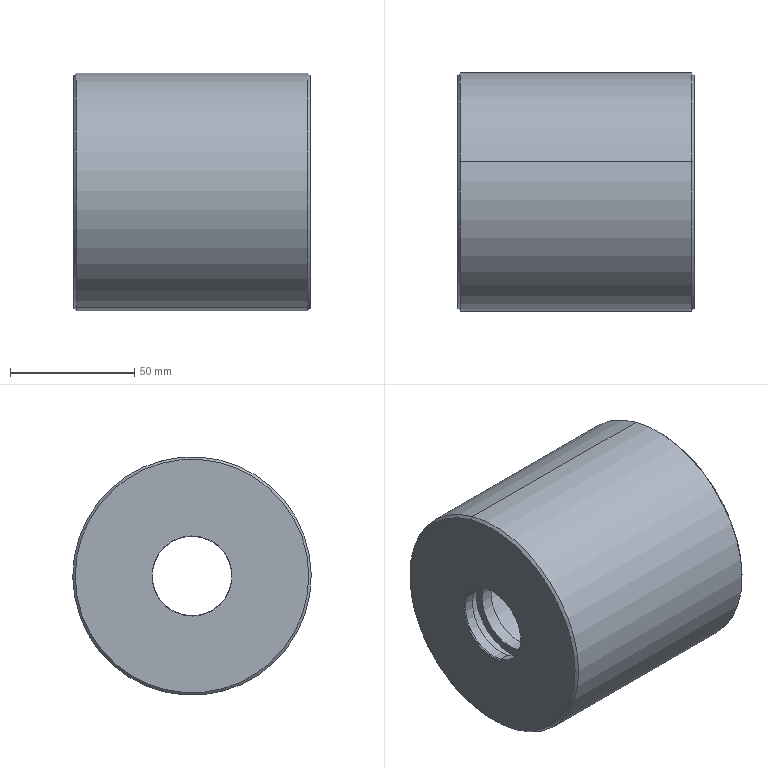Component | SolidWorks | 216InnerTubeAssembly-1_BearingSleeve1-1 | 1 solid | 37 faces | box 95 x 96 x 96 mm | volume 345909 mm3 | cylinder 18 | plane 9 | cone 8 | torus 2 | commonest cylinder face diameters 72 x6 32 x4 75 x4 39 x2 96 x2 | material Alloy Steel
build123d program:
from build123d import *


with BuildPart() as part:
    # Model → Revolve1 (revolve)
    with BuildSketch(Plane.XY):
        with BuildLine():
            ThreePointArc((17, 36), (15.586, 35.414), (15, 34))
            Line((15, 34), (15, 16))
            Line((15, 16), (10, 16))
            Line((10, 16), (10, 19.5))
            Line((10, 19.5), (4.6, 19.5))
            Line((4.6, 19.5), (4.6, 16))
            Line((4.6, 16), (0.5, 16))
            Line((0.5, 16), (0, 16.134))
            Line((0, 16.134), (0, 47))
            Line((0, 47), (1, 48))
            Line((1, 48), (94, 48))
            Line((94, 48), (95, 47))
            Line((95, 47), (95, 36.5))
            Line((95, 36.5), (94, 36))
            Line((94, 36), (90, 36))
            Line((90, 36), (90, 37.5))
            Line((90, 37.5), (87.6, 37.5))
            Line((87.6, 37.5), (87.6, 36))
            Line((87.6, 36), (82.6, 36))
            Line((82.6, 36), (82.6, 37.5))
            Line((82.6, 37.5), (80.2, 37.5))
            Line((80.2, 37.5), (80.2, 36))
            Line((80.2, 36), (17, 36))
        make_face()
    revolve(axis=Axis((119.672, 0, 0), (-1, 0, 0)))


solid = part.part

# Placed as in the assembly
solid = solid.moved(Location((826.279, 0, 0), (0, 0, 0)))
STEP:
#1=COLOUR_RGB('',0.7922,0.8196,0.9333);
#2=FILL_AREA_STYLE_COLOUR('',#1);
#3=FILL_AREA_STYLE('',(#2));
#4=SURFACE_STYLE_FILL_AREA(#3);
#5=SURFACE_SIDE_STYLE('',(#4));
#6=SURFACE_STYLE_USAGE(.BOTH.,#5);
#7=PRESENTATION_STYLE_ASSIGNMENT((#6));
#8=CARTESIAN_POINT('',(32.924,0.1615,0.6089));
#9=VERTEX_POINT('',#8);
#10=CARTESIAN_POINT('',(32.924,-0.1615,-0.6089));
#11=VERTEX_POINT('',#10);
#12=CARTESIAN_POINT('',(32.924,-0.,-0.));
#13=DIRECTION('',(1.,0.,-0.));
#14=DIRECTION('',(0.,-0.2564,-0.9666));
#15=AXIS2_PLACEMENT_3D('',#12,#13,#14);
#16=CIRCLE('',#15,0.6299);
#17=EDGE_CURVE('',#9,#11,#16,.T.);
#18=ORIENTED_EDGE('',*,*,#17,.F.);
#19=CARTESIAN_POINT('',(33.121,0.1615,0.6089));
#20=VERTEX_POINT('',#19);
#21=CARTESIAN_POINT('',(37.242,0.1615,0.6089));
#22=DIRECTION('',(1.,0.,-0.));
#23=VECTOR('',#22,39.37);
#24=LINE('',#21,#23);
#25=EDGE_CURVE('',#9,#20,#24,.T.);
#26=ORIENTED_EDGE('',*,*,#25,.T.);
#27=CARTESIAN_POINT('',(33.121,-0.1615,-0.6089));
#28=VERTEX_POINT('',#27);
#29=CARTESIAN_POINT('',(33.121,-0.,-0.));
#30=DIRECTION('',(1.,0.,-0.));
#31=DIRECTION('',(0.,-0.2564,-0.9666));
#32=AXIS2_PLACEMENT_3D('',#29,#30,#31);
#33=CIRCLE('',#32,0.6299);
#34=EDGE_CURVE('',#20,#28,#33,.T.);
#35=ORIENTED_EDGE('',*,*,#34,.T.);
#36=CARTESIAN_POINT('',(37.242,-0.1615,-0.6089));
#37=DIRECTION('',(1.,0.,-0.));
#38=VECTOR('',#37,39.37);
#39=LINE('',#36,#38);
#40=EDGE_CURVE('',#11,#28,#39,.T.);
#41=ORIENTED_EDGE('',*,*,#40,.F.);
#42=EDGE_LOOP('',(#18,#26,#35,#41));
#43=FACE_OUTER_BOUND('',#42,.T.);
#44=CARTESIAN_POINT('',(37.242,-0.,-0.));
#45=DIRECTION('',(1.,0.,-0.));
#46=DIRECTION('',(0.,-0.2564,-0.9666));
#47=AXIS2_PLACEMENT_3D('',#44,#45,#46);
#48=CYLINDRICAL_SURFACE('',#47,0.6299);
#49=ADVANCED_FACE('',(#43),#48,.F.);
#50=CARTESIAN_POINT('',(32.712,0.1969,0.742));
#51=VERTEX_POINT('',#50);
#52=CARTESIAN_POINT('',(32.712,-0.1969,-0.742));
#53=VERTEX_POINT('',#52);
#54=CARTESIAN_POINT('',(32.712,-0.,-0.));
#55=DIRECTION('',(1.,0.,-0.));
#56=DIRECTION('',(0.,-0.2564,-0.9666));
#57=AXIS2_PLACEMENT_3D('',#54,#55,#56);
#58=CIRCLE('',#57,0.7677);
#59=EDGE_CURVE('',#51,#53,#58,.T.);
#60=ORIENTED_EDGE('',*,*,#59,.F.);
#61=CARTESIAN_POINT('',(32.924,0.1969,0.742));
#62=VERTEX_POINT('',#61);
#63=CARTESIAN_POINT('',(37.242,0.1969,0.742));
#64=DIRECTION('',(1.,0.,-0.));
#65=VECTOR('',#64,39.37);
#66=LINE('',#63,#65);
#67=EDGE_CURVE('',#51,#62,#66,.T.);
#68=ORIENTED_EDGE('',*,*,#67,.T.);
#69=CARTESIAN_POINT('',(32.924,-0.1969,-0.742));
#70=VERTEX_POINT('',#69);
#71=CARTESIAN_POINT('',(32.924,-0.,-0.));
#72=DIRECTION('',(1.,0.,-0.));
#73=DIRECTION('',(0.,-0.2564,-0.9666));
#74=AXIS2_PLACEMENT_3D('',#71,#72,#73);
#75=CIRCLE('',#74,0.7677);
#76=EDGE_CURVE('',#62,#70,#75,.T.);
#77=ORIENTED_EDGE('',*,*,#76,.T.);
#78=CARTESIAN_POINT('',(37.242,-0.1969,-0.742));
#79=DIRECTION('',(1.,0.,-0.));
#80=VECTOR('',#79,39.37);
#81=LINE('',#78,#80);
#82=EDGE_CURVE('',#53,#70,#81,.T.);
#83=ORIENTED_EDGE('',*,*,#82,.F.);
#84=EDGE_LOOP('',(#60,#68,#77,#83));
#85=FACE_OUTER_BOUND('',#84,.T.);
#86=CARTESIAN_POINT('',(37.242,-0.,-0.));
#87=DIRECTION('',(1.,0.,-0.));
#88=DIRECTION('',(0.,-0.2564,-0.9666));
#89=AXIS2_PLACEMENT_3D('',#86,#87,#88);
#90=CYLINDRICAL_SURFACE('',#89,0.7677);
#91=ADVANCED_FACE('',(#85),#90,.F.);
#92=CARTESIAN_POINT('',(32.55,0.1615,0.6089));
#93=VERTEX_POINT('',#92);
#94=CARTESIAN_POINT('',(32.55,-0.1615,-0.6089));
#95=VERTEX_POINT('',#94);
#96=CARTESIAN_POINT('',(32.55,-0.,-0.));
#97=DIRECTION('',(1.,0.,-0.));
#98=DIRECTION('',(0.,-0.2564,-0.9666));
#99=AXIS2_PLACEMENT_3D('',#96,#97,#98);
#100=CIRCLE('',#99,0.6299);
#101=EDGE_CURVE('',#93,#95,#100,.T.);
#102=ORIENTED_EDGE('',*,*,#101,.F.);
#103=CARTESIAN_POINT('',(32.712,0.1615,0.6089));
#104=VERTEX_POINT('',#103);
#105=CARTESIAN_POINT('',(37.242,0.1615,0.6089));
#106=DIRECTION('',(1.,0.,-0.));
#107=VECTOR('',#106,39.37);
#108=LINE('',#105,#107);
#109=EDGE_CURVE('',#93,#104,#108,.T.);
#110=ORIENTED_EDGE('',*,*,#109,.T.);
#111=CARTESIAN_POINT('',(32.712,-0.1615,-0.6089));
#112=VERTEX_POINT('',#111);
#113=CARTESIAN_POINT('',(32.712,-0.,-0.));
#114=DIRECTION('',(1.,0.,-0.));
#115=DIRECTION('',(0.,-0.2564,-0.9666));
#116=AXIS2_PLACEMENT_3D('',#113,#114,#115);
#117=CIRCLE('',#116,0.6299);
#118=EDGE_CURVE('',#104,#112,#117,.T.);
#119=ORIENTED_EDGE('',*,*,#118,.T.);
#120=CARTESIAN_POINT('',(37.242,-0.1615,-0.6089));
#121=DIRECTION('',(1.,0.,-0.));
#122=VECTOR('',#121,39.37);
#123=LINE('',#120,#122);
#124=EDGE_CURVE('',#95,#112,#123,.T.);
#125=ORIENTED_EDGE('',*,*,#124,.F.);
#126=EDGE_LOOP('',(#102,#110,#119,#125));
#127=FACE_OUTER_BOUND('',#126,.T.);
#128=CARTESIAN_POINT('',(37.242,-0.,-0.));
#129=DIRECTION('',(1.,0.,-0.));
#130=DIRECTION('',(0.,-0.2564,-0.9666));
#131=AXIS2_PLACEMENT_3D('',#128,#129,#130);
#132=CYLINDRICAL_SURFACE('',#131,0.6299);
#133=ADVANCED_FACE('',(#127),#132,.F.);
#134=ORIENTED_EDGE('',*,*,#101,.T.);
#135=CARTESIAN_POINT('',(32.531,-0.1629,-0.614));
#136=VERTEX_POINT('',#135);
#137=CARTESIAN_POINT('',(32.55,-0.1615,-0.6089));
#138=DIRECTION('',(-0.9659,-0.06637,-0.2502));
#139=VECTOR('',#138,39.37);
#140=LINE('',#137,#139);
#141=EDGE_CURVE('',#95,#136,#140,.T.);
#142=ORIENTED_EDGE('',*,*,#141,.T.);
#143=CARTESIAN_POINT('',(32.531,0.1629,0.614));
#144=VERTEX_POINT('',#143);
#145=CARTESIAN_POINT('',(32.531,-0.,-0.));
#146=DIRECTION('',(1.,0.,-0.));
#147=DIRECTION('',(0.,-0.2564,-0.9666));
#148=AXIS2_PLACEMENT_3D('',#145,#146,#147);
#149=CIRCLE('',#148,0.6352);
#150=EDGE_CURVE('',#144,#136,#149,.T.);
#151=ORIENTED_EDGE('',*,*,#150,.F.);
#152=CARTESIAN_POINT('',(32.55,0.1615,0.6089));
#153=DIRECTION('',(-0.9659,0.06637,0.2502));
#154=VECTOR('',#153,39.37);
#155=LINE('',#152,#154);
#156=EDGE_CURVE('',#93,#144,#155,.T.);
#157=ORIENTED_EDGE('',*,*,#156,.F.);
#158=EDGE_LOOP('',(#134,#142,#151,#157));
#159=FACE_OUTER_BOUND('',#158,.T.);
#160=CARTESIAN_POINT('',(32.55,-0.,-0.));
#161=DIRECTION('',(-1.,-0.,0.));
#162=DIRECTION('',(0.,0.2564,0.9666));
#163=AXIS2_PLACEMENT_3D('',#160,#161,#162);
#164=CONICAL_SURFACE('',#163,0.6299,0.2618);
#165=ADVANCED_FACE('',(#159),#164,.F.);
#166=CARTESIAN_POINT('',(32.531,-0.4745,-1.789));
#167=VERTEX_POINT('',#166);
#168=CARTESIAN_POINT('',(32.531,0.4745,1.789));
#169=VERTEX_POINT('',#168);
#170=CARTESIAN_POINT('',(32.531,-0.,-0.));
#171=DIRECTION('',(1.,0.,-0.));
#172=DIRECTION('',(0.,-0.2564,-0.9666));
#173=AXIS2_PLACEMENT_3D('',#170,#171,#172);
#174=CIRCLE('',#173,1.85);
#175=EDGE_CURVE('',#167,#169,#174,.T.);
#176=ORIENTED_EDGE('',*,*,#175,.T.);
#177=CARTESIAN_POINT('',(32.57,0.4846,1.827));
#178=VERTEX_POINT('',#177);
#179=CARTESIAN_POINT('',(32.57,0.4846,1.827));
#180=DIRECTION('',(0.7071,0.1813,0.6835));
#181=VECTOR('',#180,39.37);
#182=LINE('',#179,#181);
#183=EDGE_CURVE('',#169,#178,#182,.T.);
#184=ORIENTED_EDGE('',*,*,#183,.T.);
#185=CARTESIAN_POINT('',(32.57,-0.4846,-1.827));
#186=VERTEX_POINT('',#185);
#187=CARTESIAN_POINT('',(32.57,-0.,-0.));
#188=DIRECTION('',(1.,0.,-0.));
#189=DIRECTION('',(0.,-0.2564,-0.9666));
#190=AXIS2_PLACEMENT_3D('',#187,#188,#189);
#191=CIRCLE('',#190,1.89);
#192=EDGE_CURVE('',#186,#178,#191,.T.);
#193=ORIENTED_EDGE('',*,*,#192,.F.);
#194=CARTESIAN_POINT('',(32.57,-0.4846,-1.827));
#195=DIRECTION('',(0.7071,-0.1813,-0.6835));
#196=VECTOR('',#195,39.37);
#197=LINE('',#194,#196);
#198=EDGE_CURVE('',#167,#186,#197,.T.);
#199=ORIENTED_EDGE('',*,*,#198,.F.);
#200=EDGE_LOOP('',(#176,#184,#193,#199));
#201=FACE_OUTER_BOUND('',#200,.T.);
#202=CARTESIAN_POINT('',(32.57,-0.,-0.));
#203=DIRECTION('',(1.,0.,-0.));
#204=DIRECTION('',(0.,-0.2564,-0.9666));
#205=AXIS2_PLACEMENT_3D('',#202,#203,#204);
#206=CONICAL_SURFACE('',#205,1.89,0.7854);
#207=ADVANCED_FACE('',(#201),#206,.T.);
#208=ORIENTED_EDGE('',*,*,#192,.T.);
#209=CARTESIAN_POINT('',(36.231,0.4846,1.827));
#210=VERTEX_POINT('',#209);
#211=CARTESIAN_POINT('',(37.242,0.4846,1.827));
#212=DIRECTION('',(1.,0.,-0.));
#213=VECTOR('',#212,39.37);
#214=LINE('',#211,#213);
#215=EDGE_CURVE('',#178,#210,#214,.T.);
#216=ORIENTED_EDGE('',*,*,#215,.T.);
#217=CARTESIAN_POINT('',(36.231,-0.4846,-1.827));
#218=VERTEX_POINT('',#217);
#219=CARTESIAN_POINT('',(36.231,-0.,-0.));
#220=DIRECTION('',(1.,0.,-0.));
#221=DIRECTION('',(0.,-0.2564,-0.9666));
#222=AXIS2_PLACEMENT_3D('',#219,#220,#221);
#223=CIRCLE('',#222,1.89);
#224=EDGE_CURVE('',#218,#210,#223,.T.);
#225=ORIENTED_EDGE('',*,*,#224,.F.);
#226=CARTESIAN_POINT('',(37.242,-0.4846,-1.827));
#227=DIRECTION('',(1.,0.,-0.));
#228=VECTOR('',#227,39.37);
#229=LINE('',#226,#228);
#230=EDGE_CURVE('',#186,#218,#229,.T.);
#231=ORIENTED_EDGE('',*,*,#230,.F.);
#232=EDGE_LOOP('',(#208,#216,#225,#231));
#233=FACE_OUTER_BOUND('',#232,.T.);
#234=CARTESIAN_POINT('',(37.242,-0.,-0.));
#235=DIRECTION('',(1.,0.,-0.));
#236=DIRECTION('',(0.,-0.2564,-0.9666));
#237=AXIS2_PLACEMENT_3D('',#234,#235,#236);
#238=CYLINDRICAL_SURFACE('',#237,1.89);
#239=ADVANCED_FACE('',(#233),#238,.T.);
#240=CARTESIAN_POINT('',(36.271,-0.4745,-1.789));
#241=VERTEX_POINT('',#240);
#242=CARTESIAN_POINT('',(36.271,0.4745,1.789));
#243=VERTEX_POINT('',#242);
#244=CARTESIAN_POINT('',(36.271,-0.,-0.));
#245=DIRECTION('',(1.,0.,-0.));
#246=DIRECTION('',(0.,-0.2564,-0.9666));
#247=AXIS2_PLACEMENT_3D('',#244,#245,#246);
#248=CIRCLE('',#247,1.85);
#249=EDGE_CURVE('',#241,#243,#248,.T.);
#250=ORIENTED_EDGE('',*,*,#249,.F.);
#251=CARTESIAN_POINT('',(36.271,-0.4745,-1.789));
#252=DIRECTION('',(-0.7071,-0.1813,-0.6835));
#253=VECTOR('',#252,39.37);
#254=LINE('',#251,#253);
#255=EDGE_CURVE('',#241,#218,#254,.T.);
#256=ORIENTED_EDGE('',*,*,#255,.T.);
#257=ORIENTED_EDGE('',*,*,#224,.T.);
#258=CARTESIAN_POINT('',(36.271,0.4745,1.789));
#259=DIRECTION('',(-0.7071,0.1813,0.6835));
#260=VECTOR('',#259,39.37);
#261=LINE('',#258,#260);
#262=EDGE_CURVE('',#243,#210,#261,.T.);
#263=ORIENTED_EDGE('',*,*,#262,.F.);
#264=EDGE_LOOP('',(#250,#256,#257,#263));
#265=FACE_OUTER_BOUND('',#264,.T.);
#266=CARTESIAN_POINT('',(36.271,-0.,-0.));
#267=DIRECTION('',(-1.,-0.,0.));
#268=DIRECTION('',(0.,0.2564,0.9666));
#269=AXIS2_PLACEMENT_3D('',#266,#267,#268);
#270=CONICAL_SURFACE('',#269,1.85,0.7854);
#271=ADVANCED_FACE('',(#265),#270,.T.);
#272=CARTESIAN_POINT('',(36.231,0.3634,1.37));
#273=VERTEX_POINT('',#272);
#274=CARTESIAN_POINT('',(36.231,-0.3634,-1.37));
#275=VERTEX_POINT('',#274);
#276=CARTESIAN_POINT('',(36.231,-0.,-0.));
#277=DIRECTION('',(1.,0.,-0.));
#278=DIRECTION('',(0.,-0.2564,-0.9666));
#279=AXIS2_PLACEMENT_3D('',#276,#277,#278);
#280=CIRCLE('',#279,1.417);
#281=EDGE_CURVE('',#273,#275,#280,.T.);
#282=ORIENTED_EDGE('',*,*,#281,.F.);
#283=CARTESIAN_POINT('',(36.271,0.3685,1.389));
#284=VERTEX_POINT('',#283);
#285=CARTESIAN_POINT('',(36.231,0.3634,1.37));
#286=DIRECTION('',(0.8944,0.1147,0.4323));
#287=VECTOR('',#286,39.37);
#288=LINE('',#285,#287);
#289=EDGE_CURVE('',#273,#284,#288,.T.);
#290=ORIENTED_EDGE('',*,*,#289,.T.);
#291=CARTESIAN_POINT('',(36.271,-0.3685,-1.389));
#292=VERTEX_POINT('',#291);
#293=CARTESIAN_POINT('',(36.271,-0.,-0.));
#294=DIRECTION('',(1.,0.,-0.));
#295=DIRECTION('',(0.,-0.2564,-0.9666));
#296=AXIS2_PLACEMENT_3D('',#293,#294,#295);
#297=CIRCLE('',#296,1.437);
#298=EDGE_CURVE('',#284,#292,#297,.T.);
#299=ORIENTED_EDGE('',*,*,#298,.T.);
#300=CARTESIAN_POINT('',(36.231,-0.3634,-1.37));
#301=DIRECTION('',(0.8944,-0.1147,-0.4323));
#302=VECTOR('',#301,39.37);
#303=LINE('',#300,#302);
#304=EDGE_CURVE('',#275,#292,#303,.T.);
#305=ORIENTED_EDGE('',*,*,#304,.F.);
#306=EDGE_LOOP('',(#282,#290,#299,#305));
#307=FACE_OUTER_BOUND('',#306,.T.);
#308=CARTESIAN_POINT('',(36.231,-0.,-0.));
#309=DIRECTION('',(1.,0.,-0.));
#310=DIRECTION('',(0.,-0.2564,-0.9666));
#311=AXIS2_PLACEMENT_3D('',#308,#309,#310);
#312=CONICAL_SURFACE('',#311,1.417,0.4636);
#313=ADVANCED_FACE('',(#307),#312,.F.);
#314=CARTESIAN_POINT('',(36.074,0.3634,1.37));
#315=VERTEX_POINT('',#314);
#316=CARTESIAN_POINT('',(36.074,-0.3634,-1.37));
#317=VERTEX_POINT('',#316);
#318=CARTESIAN_POINT('',(36.074,-0.,-0.));
#319=DIRECTION('',(1.,0.,-0.));
#320=DIRECTION('',(0.,-0.2564,-0.9666));
#321=AXIS2_PLACEMENT_3D('',#318,#319,#320);
#322=CIRCLE('',#321,1.417);
#323=EDGE_CURVE('',#315,#317,#322,.T.);
#324=ORIENTED_EDGE('',*,*,#323,.F.);
#325=CARTESIAN_POINT('',(37.242,0.3634,1.37));
#326=DIRECTION('',(1.,0.,-0.));
#327=VECTOR('',#326,39.37);
#328=LINE('',#325,#327);
#329=EDGE_CURVE('',#315,#273,#328,.T.);
#330=ORIENTED_EDGE('',*,*,#329,.T.);
#331=ORIENTED_EDGE('',*,*,#281,.T.);
#332=CARTESIAN_POINT('',(37.242,-0.3634,-1.37));
#333=DIRECTION('',(1.,0.,-0.));
#334=VECTOR('',#333,39.37);
#335=LINE('',#332,#334);
#336=EDGE_CURVE('',#317,#275,#335,.T.);
#337=ORIENTED_EDGE('',*,*,#336,.F.);
#338=EDGE_LOOP('',(#324,#330,#331,#337));
#339=FACE_OUTER_BOUND('',#338,.T.);
#340=CARTESIAN_POINT('',(37.242,-0.,-0.));
#341=DIRECTION('',(1.,0.,-0.));
#342=DIRECTION('',(0.,-0.2564,-0.9666));
#343=AXIS2_PLACEMENT_3D('',#340,#341,#342);
#344=CYLINDRICAL_SURFACE('',#343,1.417);
#345=ADVANCED_FACE('',(#339),#344,.F.);
#346=CARTESIAN_POINT('',(35.979,0.3786,1.427));
#347=VERTEX_POINT('',#346);
#348=CARTESIAN_POINT('',(35.979,-0.3786,-1.427));
#349=VERTEX_POINT('',#348);
#350=CARTESIAN_POINT('',(35.979,-0.,-0.));
#351=DIRECTION('',(1.,0.,-0.));
#352=DIRECTION('',(0.,-0.2564,-0.9666));
#353=AXIS2_PLACEMENT_3D('',#350,#351,#352);
#354=CIRCLE('',#353,1.476);
#355=EDGE_CURVE('',#347,#349,#354,.T.);
#356=ORIENTED_EDGE('',*,*,#355,.F.);
#357=CARTESIAN_POINT('',(36.074,0.3786,1.427));
#358=VERTEX_POINT('',#357);
#359=CARTESIAN_POINT('',(37.242,0.3786,1.427));
#360=DIRECTION('',(1.,0.,-0.));
#361=VECTOR('',#360,39.37);
#362=LINE('',#359,#361);
#363=EDGE_CURVE('',#347,#358,#362,.T.);
#364=ORIENTED_EDGE('',*,*,#363,.T.);
#365=CARTESIAN_POINT('',(36.074,-0.3786,-1.427));
#366=VERTEX_POINT('',#365);
#367=CARTESIAN_POINT('',(36.074,-0.,-0.));
#368=DIRECTION('',(1.,0.,-0.));
#369=DIRECTION('',(0.,-0.2564,-0.9666));
#370=AXIS2_PLACEMENT_3D('',#367,#368,#369);
#371=CIRCLE('',#370,1.476);
#372=EDGE_CURVE('',#358,#366,#371,.T.);
#373=ORIENTED_EDGE('',*,*,#372,.T.);
#374=CARTESIAN_POINT('',(37.242,-0.3786,-1.427));
#375=DIRECTION('',(1.,0.,-0.));
#376=VECTOR('',#375,39.37);
#377=LINE('',#374,#376);
#378=EDGE_CURVE('',#349,#366,#377,.T.);
#379=ORIENTED_EDGE('',*,*,#378,.F.);
#380=EDGE_LOOP('',(#356,#364,#373,#379));
#381=FACE_OUTER_BOUND('',#380,.T.);
#382=CARTESIAN_POINT('',(37.242,-0.,-0.));
#383=DIRECTION('',(1.,0.,-0.));
#384=DIRECTION('',(0.,-0.2564,-0.9666));
#385=AXIS2_PLACEMENT_3D('',#382,#383,#384);
#386=CYLINDRICAL_SURFACE('',#385,1.476);
#387=ADVANCED_FACE('',(#381),#386,.F.);
#388=CARTESIAN_POINT('',(35.783,0.3634,1.37));
#389=VERTEX_POINT('',#388);
#390=CARTESIAN_POINT('',(35.783,-0.3634,-1.37));
#391=VERTEX_POINT('',#390);
#392=CARTESIAN_POINT('',(35.783,-0.,-0.));
#393=DIRECTION('',(1.,0.,-0.));
#394=DIRECTION('',(0.,-0.2564,-0.9666));
#395=AXIS2_PLACEMENT_3D('',#392,#393,#394);
#396=CIRCLE('',#395,1.417);
#397=EDGE_CURVE('',#389,#391,#396,.T.);
#398=ORIENTED_EDGE('',*,*,#397,.F.);
#399=CARTESIAN_POINT('',(35.979,0.3634,1.37));
#400=VERTEX_POINT('',#399);
#401=CARTESIAN_POINT('',(37.242,0.3634,1.37));
#402=DIRECTION('',(1.,0.,-0.));
#403=VECTOR('',#402,39.37);
#404=LINE('',#401,#403);
#405=EDGE_CURVE('',#389,#400,#404,.T.);
#406=ORIENTED_EDGE('',*,*,#405,.T.);
#407=CARTESIAN_POINT('',(35.979,-0.3634,-1.37));
#408=VERTEX_POINT('',#407);
#409=CARTESIAN_POINT('',(35.979,-0.,-0.));
#410=DIRECTION('',(1.,0.,-0.));
#411=DIRECTION('',(0.,-0.2564,-0.9666));
#412=AXIS2_PLACEMENT_3D('',#409,#410,#411);
#413=CIRCLE('',#412,1.417);
#414=EDGE_CURVE('',#400,#408,#413,.T.);
#415=ORIENTED_EDGE('',*,*,#414,.T.);
#416=CARTESIAN_POINT('',(37.242,-0.3634,-1.37));
#417=DIRECTION('',(1.,0.,-0.));
#418=VECTOR('',#417,39.37);
#419=LINE('',#416,#418);
#420=EDGE_CURVE('',#391,#408,#419,.T.);
#421=ORIENTED_EDGE('',*,*,#420,.F.);
#422=EDGE_LOOP('',(#398,#406,#415,#421));
#423=FACE_OUTER_BOUND('',#422,.T.);
#424=CARTESIAN_POINT('',(37.242,-0.,-0.));
#425=DIRECTION('',(1.,0.,-0.));
#426=DIRECTION('',(0.,-0.2564,-0.9666));
#427=AXIS2_PLACEMENT_3D('',#424,#425,#426);
#428=CYLINDRICAL_SURFACE('',#427,1.417);
#429=ADVANCED_FACE('',(#423),#428,.F.);
#430=CARTESIAN_POINT('',(35.688,0.3786,1.427));
#431=VERTEX_POINT('',#430);
#432=CARTESIAN_POINT('',(35.688,-0.3786,-1.427));
#433=VERTEX_POINT('',#432);
#434=CARTESIAN_POINT('',(35.688,-0.,-0.));
#435=DIRECTION('',(1.,0.,-0.));
#436=DIRECTION('',(0.,-0.2564,-0.9666));
#437=AXIS2_PLACEMENT_3D('',#434,#435,#436);
#438=CIRCLE('',#437,1.476);
#439=EDGE_CURVE('',#431,#433,#438,.T.);
#440=ORIENTED_EDGE('',*,*,#439,.F.);
#441=CARTESIAN_POINT('',(35.783,0.3786,1.427));
#442=VERTEX_POINT('',#441);
#443=CARTESIAN_POINT('',(37.242,0.3786,1.427));
#444=DIRECTION('',(1.,0.,-0.));
#445=VECTOR('',#444,39.37);
#446=LINE('',#443,#445);
#447=EDGE_CURVE('',#431,#442,#446,.T.);
#448=ORIENTED_EDGE('',*,*,#447,.T.);
#449=CARTESIAN_POINT('',(35.783,-0.3786,-1.427));
#450=VERTEX_POINT('',#449);
#451=CARTESIAN_POINT('',(35.783,-0.,-0.));
#452=DIRECTION('',(1.,0.,-0.));
#453=DIRECTION('',(0.,-0.2564,-0.9666));
#454=AXIS2_PLACEMENT_3D('',#451,#452,#453);
#455=CIRCLE('',#454,1.476);
#456=EDGE_CURVE('',#442,#450,#455,.T.);
#457=ORIENTED_EDGE('',*,*,#456,.T.);
#458=CARTESIAN_POINT('',(37.242,-0.3786,-1.427));
#459=DIRECTION('',(1.,0.,-0.));
#460=VECTOR('',#459,39.37);
#461=LINE('',#458,#460);
#462=EDGE_CURVE('',#433,#450,#461,.T.);
#463=ORIENTED_EDGE('',*,*,#462,.F.);
#464=EDGE_LOOP('',(#440,#448,#457,#463));
#465=FACE_OUTER_BOUND('',#464,.T.);
#466=CARTESIAN_POINT('',(37.242,-0.,-0.));
#467=DIRECTION('',(1.,0.,-0.));
#468=DIRECTION('',(0.,-0.2564,-0.9666));
#469=AXIS2_PLACEMENT_3D('',#466,#467,#468);
#470=CYLINDRICAL_SURFACE('',#469,1.476);
#471=ADVANCED_FACE('',(#465),#470,.F.);
#472=CARTESIAN_POINT('',(33.2,0.3634,1.37));
#473=VERTEX_POINT('',#472);
#474=CARTESIAN_POINT('',(33.2,-0.3634,-1.37));
#475=VERTEX_POINT('',#474);
#476=CARTESIAN_POINT('',(33.2,-0.,-0.));
#477=DIRECTION('',(1.,0.,-0.));
#478=DIRECTION('',(0.,-0.2564,-0.9666));
#479=AXIS2_PLACEMENT_3D('',#476,#477,#478);
#480=CIRCLE('',#479,1.417);
#481=EDGE_CURVE('',#473,#475,#480,.T.);
#482=ORIENTED_EDGE('',*,*,#481,.F.);
#483=CARTESIAN_POINT('',(35.688,0.3634,1.37));
#484=VERTEX_POINT('',#483);
#485=CARTESIAN_POINT('',(37.242,0.3634,1.37));
#486=DIRECTION('',(1.,0.,-0.));
#487=VECTOR('',#486,39.37);
#488=LINE('',#485,#487);
#489=EDGE_CURVE('',#473,#484,#488,.T.);
#490=ORIENTED_EDGE('',*,*,#489,.T.);
#491=CARTESIAN_POINT('',(35.688,-0.3634,-1.37));
#492=VERTEX_POINT('',#491);
#493=CARTESIAN_POINT('',(35.688,-0.,-0.));
#494=DIRECTION('',(1.,0.,-0.));
#495=DIRECTION('',(0.,-0.2564,-0.9666));
#496=AXIS2_PLACEMENT_3D('',#493,#494,#495);
#497=CIRCLE('',#496,1.417);
#498=EDGE_CURVE('',#484,#492,#497,.T.);
#499=ORIENTED_EDGE('',*,*,#498,.T.);
#500=CARTESIAN_POINT('',(37.242,-0.3634,-1.37));
#501=DIRECTION('',(1.,0.,-0.));
#502=VECTOR('',#501,39.37);
#503=LINE('',#500,#502);
#504=EDGE_CURVE('',#475,#492,#503,.T.);
#505=ORIENTED_EDGE('',*,*,#504,.F.);
#506=EDGE_LOOP('',(#482,#490,#499,#505));
#507=FACE_OUTER_BOUND('',#506,.T.);
#508=CARTESIAN_POINT('',(37.242,-0.,-0.));
#509=DIRECTION('',(1.,0.,-0.));
#510=DIRECTION('',(0.,-0.2564,-0.9666));
#511=AXIS2_PLACEMENT_3D('',#508,#509,#510);
#512=CYLINDRICAL_SURFACE('',#511,1.417);
#513=ADVANCED_FACE('',(#507),#512,.F.);
#514=CARTESIAN_POINT('',(33.121,0.3433,1.294));
#515=VERTEX_POINT('',#514);
#516=CARTESIAN_POINT('',(33.121,-0.3433,-1.294));
#517=VERTEX_POINT('',#516);
#518=CARTESIAN_POINT('',(33.121,-0.,-0.));
#519=DIRECTION('',(1.,0.,-0.));
#520=DIRECTION('',(0.,-0.2564,-0.9666));
#521=AXIS2_PLACEMENT_3D('',#518,#519,#520);
#522=CIRCLE('',#521,1.339);
#523=EDGE_CURVE('',#515,#517,#522,.T.);
#524=ORIENTED_EDGE('',*,*,#523,.F.);
#525=CARTESIAN_POINT('',(33.2,0.3433,1.294));
#526=DIRECTION('',(-0.,0.9666,-0.2564));
#527=DIRECTION('',(0.,0.2564,0.9666));
#528=AXIS2_PLACEMENT_3D('',#525,#526,#527);
#529=CIRCLE('',#528,0.07874);
#530=EDGE_CURVE('',#515,#473,#529,.T.);
#531=ORIENTED_EDGE('',*,*,#530,.T.);
#532=ORIENTED_EDGE('',*,*,#481,.T.);
#533=CARTESIAN_POINT('',(33.2,-0.3433,-1.294));
#534=DIRECTION('',(0.,-0.9666,0.2564));
#535=DIRECTION('',(0.,-0.2564,-0.9666));
#536=AXIS2_PLACEMENT_3D('',#533,#534,#535);
#537=CIRCLE('',#536,0.07874);
#538=EDGE_CURVE('',#517,#475,#537,.T.);
#539=ORIENTED_EDGE('',*,*,#538,.F.);
#540=EDGE_LOOP('',(#524,#531,#532,#539));
#541=FACE_OUTER_BOUND('',#540,.T.);
#542=CARTESIAN_POINT('',(33.2,-0.,-0.));
#543=DIRECTION('',(1.,0.,-0.));
#544=DIRECTION('',(0.,-0.2564,-0.9666));
#545=AXIS2_PLACEMENT_3D('',#542,#543,#544);
#546=TOROIDAL_SURFACE('',#545,1.339,0.07874);
#547=ADVANCED_FACE('',(#541),#546,.F.);
#548=ORIENTED_EDGE('',*,*,#530,.F.);
#549=CARTESIAN_POINT('',(33.121,-0.,-0.));
#550=DIRECTION('',(1.,0.,-0.));
#551=DIRECTION('',(0.,-0.2564,-0.9666));
#552=AXIS2_PLACEMENT_3D('',#549,#550,#551);
#553=CIRCLE('',#552,1.339);
#554=EDGE_CURVE('',#517,#515,#553,.T.);
#555=ORIENTED_EDGE('',*,*,#554,.F.);
#556=ORIENTED_EDGE('',*,*,#538,.T.);
#557=CARTESIAN_POINT('',(33.2,-0.,-0.));
#558=DIRECTION('',(1.,0.,-0.));
#559=DIRECTION('',(0.,-0.2564,-0.9666));
#560=AXIS2_PLACEMENT_3D('',#557,#558,#559);
#561=CIRCLE('',#560,1.417);
#562=EDGE_CURVE('',#475,#473,#561,.T.);
#563=ORIENTED_EDGE('',*,*,#562,.T.);
#564=EDGE_LOOP('',(#548,#555,#556,#563));
#565=FACE_OUTER_BOUND('',#564,.T.);
#566=CARTESIAN_POINT('',(33.2,-0.,-0.));
#567=DIRECTION('',(1.,0.,-0.));
#568=DIRECTION('',(0.,-0.2564,-0.9666));
#569=AXIS2_PLACEMENT_3D('',#566,#567,#568);
#570=TOROIDAL_SURFACE('',#569,1.339,0.07874);
#571=ADVANCED_FACE('',(#565),#570,.F.);
#572=ORIENTED_EDGE('',*,*,#489,.F.);
#573=ORIENTED_EDGE('',*,*,#562,.F.);
#574=ORIENTED_EDGE('',*,*,#504,.T.);
#575=CARTESIAN_POINT('',(35.688,-0.,-0.));
#576=DIRECTION('',(1.,0.,-0.));
#577=DIRECTION('',(0.,-0.2564,-0.9666));
#578=AXIS2_PLACEMENT_3D('',#575,#576,#577);
#579=CIRCLE('',#578,1.417);
#580=EDGE_CURVE('',#492,#484,#579,.T.);
#581=ORIENTED_EDGE('',*,*,#580,.T.);
#582=EDGE_LOOP('',(#572,#573,#574,#581));
#583=FACE_OUTER_BOUND('',#582,.T.);
#584=CARTESIAN_POINT('',(37.242,-0.,-0.));
#585=DIRECTION('',(1.,0.,-0.));
#586=DIRECTION('',(0.,-0.2564,-0.9666));
#587=AXIS2_PLACEMENT_3D('',#584,#585,#586);
#588=CYLINDRICAL_SURFACE('',#587,1.417);
#589=ADVANCED_FACE('',(#583),#588,.F.);
#590=ORIENTED_EDGE('',*,*,#580,.F.);
#591=ORIENTED_EDGE('',*,*,#498,.F.);
#592=EDGE_LOOP('',(#590,#591));
#593=FACE_BOUND('',#592,.T.);
#594=CARTESIAN_POINT('',(35.688,-0.,-0.));
#595=DIRECTION('',(1.,0.,-0.));
#596=DIRECTION('',(0.,-0.2564,-0.9666));
#597=AXIS2_PLACEMENT_3D('',#594,#595,#596);
#598=CIRCLE('',#597,1.476);
#599=EDGE_CURVE('',#433,#431,#598,.T.);
#600=ORIENTED_EDGE('',*,*,#599,.T.);
#601=ORIENTED_EDGE('',*,*,#439,.T.);
#602=EDGE_LOOP('',(#600,#601));
#603=FACE_OUTER_BOUND('',#602,.T.);
#604=CARTESIAN_POINT('',(35.688,-0.,-0.));
#605=DIRECTION('',(-1.,-0.,0.));
#606=DIRECTION('',(-0.,0.2564,0.9666));
#607=AXIS2_PLACEMENT_3D('',#604,#605,#606);
#608=PLANE('',#607);
#609=ADVANCED_FACE('',(#593,#603),#608,.F.);
#610=ORIENTED_EDGE('',*,*,#447,.F.);
#611=ORIENTED_EDGE('',*,*,#599,.F.);
#612=ORIENTED_EDGE('',*,*,#462,.T.);
#613=CARTESIAN_POINT('',(35.783,-0.,-0.));
#614=DIRECTION('',(1.,0.,-0.));
#615=DIRECTION('',(0.,-0.2564,-0.9666));
#616=AXIS2_PLACEMENT_3D('',#613,#614,#615);
#617=CIRCLE('',#616,1.476);
#618=EDGE_CURVE('',#450,#442,#617,.T.);
#619=ORIENTED_EDGE('',*,*,#618,.T.);
#620=EDGE_LOOP('',(#610,#611,#612,#619));
#621=FACE_OUTER_BOUND('',#620,.T.);
#622=CARTESIAN_POINT('',(37.242,-0.,-0.));
#623=DIRECTION('',(1.,0.,-0.));
#624=DIRECTION('',(0.,-0.2564,-0.9666));
#625=AXIS2_PLACEMENT_3D('',#622,#623,#624);
#626=CYLINDRICAL_SURFACE('',#625,1.476);
#627=ADVANCED_FACE('',(#621),#626,.F.);
#628=ORIENTED_EDGE('',*,*,#618,.F.);
#629=ORIENTED_EDGE('',*,*,#456,.F.);
#630=EDGE_LOOP('',(#628,#629));
#631=FACE_OUTER_BOUND('',#630,.T.);
#632=CARTESIAN_POINT('',(35.783,-0.,-0.));
#633=DIRECTION('',(1.,0.,-0.));
#634=DIRECTION('',(0.,-0.2564,-0.9666));
#635=AXIS2_PLACEMENT_3D('',#632,#633,#634);
#636=CIRCLE('',#635,1.417);
#637=EDGE_CURVE('',#391,#389,#636,.T.);
#638=ORIENTED_EDGE('',*,*,#637,.T.);
#639=ORIENTED_EDGE('',*,*,#397,.T.);
#640=EDGE_LOOP('',(#638,#639));
#641=FACE_BOUND('',#640,.T.);
#642=CARTESIAN_POINT('',(35.783,-0.,-0.));
#643=DIRECTION('',(1.,0.,-0.));
#644=DIRECTION('',(0.,-0.2564,-0.9666));
#645=AXIS2_PLACEMENT_3D('',#642,#643,#644);
#646=PLANE('',#645);
#647=ADVANCED_FACE('',(#631,#641),#646,.F.);
#648=ORIENTED_EDGE('',*,*,#405,.F.);
#649=ORIENTED_EDGE('',*,*,#637,.F.);
#650=ORIENTED_EDGE('',*,*,#420,.T.);
#651=CARTESIAN_POINT('',(35.979,-0.,-0.));
#652=DIRECTION('',(1.,0.,-0.));
#653=DIRECTION('',(0.,-0.2564,-0.9666));
#654=AXIS2_PLACEMENT_3D('',#651,#652,#653);
#655=CIRCLE('',#654,1.417);
#656=EDGE_CURVE('',#408,#400,#655,.T.);
#657=ORIENTED_EDGE('',*,*,#656,.T.);
#658=EDGE_LOOP('',(#648,#649,#650,#657));
#659=FACE_OUTER_BOUND('',#658,.T.);
#660=CARTESIAN_POINT('',(37.242,-0.,-0.));
#661=DIRECTION('',(1.,0.,-0.));
#662=DIRECTION('',(0.,-0.2564,-0.9666));
#663=AXIS2_PLACEMENT_3D('',#660,#661,#662);
#664=CYLINDRICAL_SURFACE('',#663,1.417);
#665=ADVANCED_FACE('',(#659),#664,.F.);
#666=ORIENTED_EDGE('',*,*,#656,.F.);
#667=ORIENTED_EDGE('',*,*,#414,.F.);
#668=EDGE_LOOP('',(#666,#667));
#669=FACE_BOUND('',#668,.T.);
#670=CARTESIAN_POINT('',(35.979,-0.,-0.));
#671=DIRECTION('',(1.,0.,-0.));
#672=DIRECTION('',(0.,-0.2564,-0.9666));
#673=AXIS2_PLACEMENT_3D('',#670,#671,#672);
#674=CIRCLE('',#673,1.476);
#675=EDGE_CURVE('',#349,#347,#674,.T.);
#676=ORIENTED_EDGE('',*,*,#675,.T.);
#677=ORIENTED_EDGE('',*,*,#355,.T.);
#678=EDGE_LOOP('',(#676,#677));
#679=FACE_OUTER_BOUND('',#678,.T.);
#680=CARTESIAN_POINT('',(35.979,-0.,-0.));
#681=DIRECTION('',(-1.,-0.,0.));
#682=DIRECTION('',(-0.,0.2564,0.9666));
#683=AXIS2_PLACEMENT_3D('',#680,#681,#682);
#684=PLANE('',#683);
#685=ADVANCED_FACE('',(#669,#679),#684,.F.);
#686=ORIENTED_EDGE('',*,*,#363,.F.);
#687=ORIENTED_EDGE('',*,*,#675,.F.);
#688=ORIENTED_EDGE('',*,*,#378,.T.);
#689=CARTESIAN_POINT('',(36.074,-0.,-0.));
#690=DIRECTION('',(1.,0.,-0.));
#691=DIRECTION('',(0.,-0.2564,-0.9666));
#692=AXIS2_PLACEMENT_3D('',#689,#690,#691);
#693=CIRCLE('',#692,1.476);
#694=EDGE_CURVE('',#366,#358,#693,.T.);
#695=ORIENTED_EDGE('',*,*,#694,.T.);
#696=EDGE_LOOP('',(#686,#687,#688,#695));
#697=FACE_OUTER_BOUND('',#696,.T.);
#698=CARTESIAN_POINT('',(37.242,-0.,-0.));
#699=DIRECTION('',(1.,0.,-0.));
#700=DIRECTION('',(0.,-0.2564,-0.9666));
#701=AXIS2_PLACEMENT_3D('',#698,#699,#700);
#702=CYLINDRICAL_SURFACE('',#701,1.476);
#703=ADVANCED_FACE('',(#697),#702,.F.);
#704=ORIENTED_EDGE('',*,*,#694,.F.);
#705=ORIENTED_EDGE('',*,*,#372,.F.);
#706=EDGE_LOOP('',(#704,#705));
#707=FACE_OUTER_BOUND('',#706,.T.);
#708=CARTESIAN_POINT('',(36.074,-0.,-0.));
#709=DIRECTION('',(1.,0.,-0.));
#710=DIRECTION('',(0.,-0.2564,-0.9666));
#711=AXIS2_PLACEMENT_3D('',#708,#709,#710);
#712=CIRCLE('',#711,1.417);
#713=EDGE_CURVE('',#317,#315,#712,.T.);
#714=ORIENTED_EDGE('',*,*,#713,.T.);
#715=ORIENTED_EDGE('',*,*,#323,.T.);
#716=EDGE_LOOP('',(#714,#715));
#717=FACE_BOUND('',#716,.T.);
#718=CARTESIAN_POINT('',(36.074,-0.,-0.));
#719=DIRECTION('',(1.,0.,-0.));
#720=DIRECTION('',(0.,-0.2564,-0.9666));
#721=AXIS2_PLACEMENT_3D('',#718,#719,#720);
#722=PLANE('',#721);
#723=ADVANCED_FACE('',(#707,#717),#722,.F.);
#724=ORIENTED_EDGE('',*,*,#329,.F.);
#725=ORIENTED_EDGE('',*,*,#713,.F.);
#726=ORIENTED_EDGE('',*,*,#336,.T.);
#727=CARTESIAN_POINT('',(36.231,-0.,-0.));
#728=DIRECTION('',(1.,0.,-0.));
#729=DIRECTION('',(0.,-0.2564,-0.9666));
#730=AXIS2_PLACEMENT_3D('',#727,#728,#729);
#731=CIRCLE('',#730,1.417);
#732=EDGE_CURVE('',#275,#273,#731,.T.);
#733=ORIENTED_EDGE('',*,*,#732,.T.);
#734=EDGE_LOOP('',(#724,#725,#726,#733));
#735=FACE_OUTER_BOUND('',#734,.T.);
#736=CARTESIAN_POINT('',(37.242,-0.,-0.));
#737=DIRECTION('',(1.,0.,-0.));
#738=DIRECTION('',(0.,-0.2564,-0.9666));
#739=AXIS2_PLACEMENT_3D('',#736,#737,#738);
#740=CYLINDRICAL_SURFACE('',#739,1.417);
#741=ADVANCED_FACE('',(#735),#740,.F.);
#742=ORIENTED_EDGE('',*,*,#289,.F.);
#743=ORIENTED_EDGE('',*,*,#732,.F.);
#744=ORIENTED_EDGE('',*,*,#304,.T.);
#745=CARTESIAN_POINT('',(36.271,-0.,-0.));
#746=DIRECTION('',(1.,0.,-0.));
#747=DIRECTION('',(0.,-0.2564,-0.9666));
#748=AXIS2_PLACEMENT_3D('',#745,#746,#747);
#749=CIRCLE('',#748,1.437);
#750=EDGE_CURVE('',#292,#284,#749,.T.);
#751=ORIENTED_EDGE('',*,*,#750,.T.);
#752=EDGE_LOOP('',(#742,#743,#744,#751));
#753=FACE_OUTER_BOUND('',#752,.T.);
#754=CARTESIAN_POINT('',(36.231,-0.,-0.));
#755=DIRECTION('',(1.,0.,-0.));
#756=DIRECTION('',(0.,-0.2564,-0.9666));
#757=AXIS2_PLACEMENT_3D('',#754,#755,#756);
#758=CONICAL_SURFACE('',#757,1.417,0.4636);
#759=ADVANCED_FACE('',(#753),#758,.F.);
#760=CARTESIAN_POINT('',(36.271,-0.,-0.));
#761=DIRECTION('',(1.,0.,-0.));
#762=DIRECTION('',(0.,-0.2564,-0.9666));
#763=AXIS2_PLACEMENT_3D('',#760,#761,#762);
#764=CIRCLE('',#763,1.85);
#765=EDGE_CURVE('',#243,#241,#764,.T.);
#766=ORIENTED_EDGE('',*,*,#765,.T.);
#767=ORIENTED_EDGE('',*,*,#249,.T.);
#768=EDGE_LOOP('',(#766,#767));
#769=FACE_OUTER_BOUND('',#768,.T.);
#770=ORIENTED_EDGE('',*,*,#750,.F.);
#771=ORIENTED_EDGE('',*,*,#298,.F.);
#772=EDGE_LOOP('',(#770,#771));
#773=FACE_BOUND('',#772,.T.);
#774=CARTESIAN_POINT('',(36.271,-0.,-0.));
#775=DIRECTION('',(1.,0.,-0.));
#776=DIRECTION('',(0.,-0.2564,-0.9666));
#777=AXIS2_PLACEMENT_3D('',#774,#775,#776);
#778=PLANE('',#777);
#779=ADVANCED_FACE('',(#769,#773),#778,.T.);
#780=ORIENTED_EDGE('',*,*,#255,.F.);
#781=ORIENTED_EDGE('',*,*,#765,.F.);
#782=ORIENTED_EDGE('',*,*,#262,.T.);
#783=CARTESIAN_POINT('',(36.231,-0.,-0.));
#784=DIRECTION('',(1.,0.,-0.));
#785=DIRECTION('',(0.,-0.2564,-0.9666));
#786=AXIS2_PLACEMENT_3D('',#783,#784,#785);
#787=CIRCLE('',#786,1.89);
#788=EDGE_CURVE('',#210,#218,#787,.T.);
#789=ORIENTED_EDGE('',*,*,#788,.T.);
#790=EDGE_LOOP('',(#780,#781,#782,#789));
#791=FACE_OUTER_BOUND('',#790,.T.);
#792=CARTESIAN_POINT('',(36.271,-0.,-0.));
#793=DIRECTION('',(-1.,-0.,0.));
#794=DIRECTION('',(0.,0.2564,0.9666));
#795=AXIS2_PLACEMENT_3D('',#792,#793,#794);
#796=CONICAL_SURFACE('',#795,1.85,0.7854);
#797=ADVANCED_FACE('',(#791),#796,.T.);
#798=ORIENTED_EDGE('',*,*,#215,.F.);
#799=CARTESIAN_POINT('',(32.57,-0.,-0.));
#800=DIRECTION('',(1.,0.,-0.));
#801=DIRECTION('',(0.,-0.2564,-0.9666));
#802=AXIS2_PLACEMENT_3D('',#799,#800,#801);
#803=CIRCLE('',#802,1.89);
#804=EDGE_CURVE('',#178,#186,#803,.T.);
#805=ORIENTED_EDGE('',*,*,#804,.T.);
#806=ORIENTED_EDGE('',*,*,#230,.T.);
#807=ORIENTED_EDGE('',*,*,#788,.F.);
#808=EDGE_LOOP('',(#798,#805,#806,#807));
#809=FACE_OUTER_BOUND('',#808,.T.);
#810=CARTESIAN_POINT('',(37.242,-0.,-0.));
#811=DIRECTION('',(1.,0.,-0.));
#812=DIRECTION('',(0.,-0.2564,-0.9666));
#813=AXIS2_PLACEMENT_3D('',#810,#811,#812);
#814=CYLINDRICAL_SURFACE('',#813,1.89);
#815=ADVANCED_FACE('',(#809),#814,.T.);
#816=ORIENTED_EDGE('',*,*,#183,.F.);
#817=CARTESIAN_POINT('',(32.531,-0.,-0.));
#818=DIRECTION('',(1.,0.,-0.));
#819=DIRECTION('',(0.,-0.2564,-0.9666));
#820=AXIS2_PLACEMENT_3D('',#817,#818,#819);
#821=CIRCLE('',#820,1.85);
#822=EDGE_CURVE('',#169,#167,#821,.T.);
#823=ORIENTED_EDGE('',*,*,#822,.T.);
#824=ORIENTED_EDGE('',*,*,#198,.T.);
#825=ORIENTED_EDGE('',*,*,#804,.F.);
#826=EDGE_LOOP('',(#816,#823,#824,#825));
#827=FACE_OUTER_BOUND('',#826,.T.);
#828=CARTESIAN_POINT('',(32.57,-0.,-0.));
#829=DIRECTION('',(1.,0.,-0.));
#830=DIRECTION('',(0.,-0.2564,-0.9666));
#831=AXIS2_PLACEMENT_3D('',#828,#829,#830);
#832=CONICAL_SURFACE('',#831,1.89,0.7854);
#833=ADVANCED_FACE('',(#827),#832,.T.);
#834=ORIENTED_EDGE('',*,*,#150,.T.);
#835=CARTESIAN_POINT('',(32.531,-0.,-0.));
#836=DIRECTION('',(1.,0.,-0.));
#837=DIRECTION('',(0.,-0.2564,-0.9666));
#838=AXIS2_PLACEMENT_3D('',#835,#836,#837);
#839=CIRCLE('',#838,0.6352);
#840=EDGE_CURVE('',#136,#144,#839,.T.);
#841=ORIENTED_EDGE('',*,*,#840,.T.);
#842=EDGE_LOOP('',(#834,#841));
#843=FACE_BOUND('',#842,.T.);
#844=ORIENTED_EDGE('',*,*,#175,.F.);
#845=ORIENTED_EDGE('',*,*,#822,.F.);
#846=EDGE_LOOP('',(#844,#845));
#847=FACE_OUTER_BOUND('',#846,.T.);
#848=CARTESIAN_POINT('',(32.531,-0.,-0.));
#849=DIRECTION('',(-1.,-0.,0.));
#850=DIRECTION('',(-0.,0.2564,0.9666));
#851=AXIS2_PLACEMENT_3D('',#848,#849,#850);
#852=PLANE('',#851);
#853=ADVANCED_FACE('',(#843,#847),#852,.T.);
#854=ORIENTED_EDGE('',*,*,#141,.F.);
#855=CARTESIAN_POINT('',(32.55,-0.,-0.));
#856=DIRECTION('',(1.,0.,-0.));
#857=DIRECTION('',(0.,-0.2564,-0.9666));
#858=AXIS2_PLACEMENT_3D('',#855,#856,#857);
#859=CIRCLE('',#858,0.6299);
#860=EDGE_CURVE('',#95,#93,#859,.T.);
#861=ORIENTED_EDGE('',*,*,#860,.T.);
#862=ORIENTED_EDGE('',*,*,#156,.T.);
#863=ORIENTED_EDGE('',*,*,#840,.F.);
#864=EDGE_LOOP('',(#854,#861,#862,#863));
#865=FACE_OUTER_BOUND('',#864,.T.);
#866=CARTESIAN_POINT('',(32.55,-0.,-0.));
#867=DIRECTION('',(-1.,-0.,0.));
#868=DIRECTION('',(0.,0.2564,0.9666));
#869=AXIS2_PLACEMENT_3D('',#866,#867,#868);
#870=CONICAL_SURFACE('',#869,0.6299,0.2618);
#871=ADVANCED_FACE('',(#865),#870,.F.);
#872=ORIENTED_EDGE('',*,*,#109,.F.);
#873=ORIENTED_EDGE('',*,*,#860,.F.);
#874=ORIENTED_EDGE('',*,*,#124,.T.);
#875=CARTESIAN_POINT('',(32.712,-0.,-0.));
#876=DIRECTION('',(1.,0.,-0.));
#877=DIRECTION('',(0.,-0.2564,-0.9666));
#878=AXIS2_PLACEMENT_3D('',#875,#876,#877);
#879=CIRCLE('',#878,0.6299);
#880=EDGE_CURVE('',#112,#104,#879,.T.);
#881=ORIENTED_EDGE('',*,*,#880,.T.);
#882=EDGE_LOOP('',(#872,#873,#874,#881));
#883=FACE_OUTER_BOUND('',#882,.T.);
#884=CARTESIAN_POINT('',(37.242,-0.,-0.));
#885=DIRECTION('',(1.,0.,-0.));
#886=DIRECTION('',(0.,-0.2564,-0.9666));
#887=AXIS2_PLACEMENT_3D('',#884,#885,#886);
#888=CYLINDRICAL_SURFACE('',#887,0.6299);
#889=ADVANCED_FACE('',(#883),#888,.F.);
#890=ORIENTED_EDGE('',*,*,#880,.F.);
#891=ORIENTED_EDGE('',*,*,#118,.F.);
#892=EDGE_LOOP('',(#890,#891));
#893=FACE_BOUND('',#892,.T.);
#894=CARTESIAN_POINT('',(32.712,-0.,-0.));
#895=DIRECTION('',(1.,0.,-0.));
#896=DIRECTION('',(0.,-0.2564,-0.9666));
#897=AXIS2_PLACEMENT_3D('',#894,#895,#896);
#898=CIRCLE('',#897,0.7677);
#899=EDGE_CURVE('',#53,#51,#898,.T.);
#900=ORIENTED_EDGE('',*,*,#899,.T.);
#901=ORIENTED_EDGE('',*,*,#59,.T.);
#902=EDGE_LOOP('',(#900,#901));
#903=FACE_OUTER_BOUND('',#902,.T.);
#904=CARTESIAN_POINT('',(32.712,-0.,-0.));
#905=DIRECTION('',(-1.,-0.,0.));
#906=DIRECTION('',(-0.,0.2564,0.9666));
#907=AXIS2_PLACEMENT_3D('',#904,#905,#906);
#908=PLANE('',#907);
#909=ADVANCED_FACE('',(#893,#903),#908,.F.);
#910=ORIENTED_EDGE('',*,*,#67,.F.);
#911=ORIENTED_EDGE('',*,*,#899,.F.);
#912=ORIENTED_EDGE('',*,*,#82,.T.);
#913=CARTESIAN_POINT('',(32.924,-0.,-0.));
#914=DIRECTION('',(1.,0.,-0.));
#915=DIRECTION('',(0.,-0.2564,-0.9666));
#916=AXIS2_PLACEMENT_3D('',#913,#914,#915);
#917=CIRCLE('',#916,0.7677);
#918=EDGE_CURVE('',#70,#62,#917,.T.);
#919=ORIENTED_EDGE('',*,*,#918,.T.);
#920=EDGE_LOOP('',(#910,#911,#912,#919));
#921=FACE_OUTER_BOUND('',#920,.T.);
#922=CARTESIAN_POINT('',(37.242,-0.,-0.));
#923=DIRECTION('',(1.,0.,-0.));
#924=DIRECTION('',(0.,-0.2564,-0.9666));
#925=AXIS2_PLACEMENT_3D('',#922,#923,#924);
#926=CYLINDRICAL_SURFACE('',#925,0.7677);
#927=ADVANCED_FACE('',(#921),#926,.F.);
#928=ORIENTED_EDGE('',*,*,#918,.F.);
#929=ORIENTED_EDGE('',*,*,#76,.F.);
#930=EDGE_LOOP('',(#928,#929));
#931=FACE_OUTER_BOUND('',#930,.T.);
#932=CARTESIAN_POINT('',(32.924,-0.,-0.));
#933=DIRECTION('',(1.,0.,-0.));
#934=DIRECTION('',(0.,-0.2564,-0.9666));
#935=AXIS2_PLACEMENT_3D('',#932,#933,#934);
#936=CIRCLE('',#935,0.6299);
#937=EDGE_CURVE('',#11,#9,#936,.T.);
#938=ORIENTED_EDGE('',*,*,#937,.T.);
#939=ORIENTED_EDGE('',*,*,#17,.T.);
#940=EDGE_LOOP('',(#938,#939));
#941=FACE_BOUND('',#940,.T.);
#942=CARTESIAN_POINT('',(32.924,-0.,-0.));
#943=DIRECTION('',(1.,0.,-0.));
#944=DIRECTION('',(0.,-0.2564,-0.9666));
#945=AXIS2_PLACEMENT_3D('',#942,#943,#944);
#946=PLANE('',#945);
#947=ADVANCED_FACE('',(#931,#941),#946,.F.);
#948=ORIENTED_EDGE('',*,*,#25,.F.);
#949=ORIENTED_EDGE('',*,*,#937,.F.);
#950=ORIENTED_EDGE('',*,*,#40,.T.);
#951=CARTESIAN_POINT('',(33.121,-0.,-0.));
#952=DIRECTION('',(1.,0.,-0.));
#953=DIRECTION('',(0.,-0.2564,-0.9666));
#954=AXIS2_PLACEMENT_3D('',#951,#952,#953);
#955=CIRCLE('',#954,0.6299);
#956=EDGE_CURVE('',#28,#20,#955,.T.);
#957=ORIENTED_EDGE('',*,*,#956,.T.);
#958=EDGE_LOOP('',(#948,#949,#950,#957));
#959=FACE_OUTER_BOUND('',#958,.T.);
#960=CARTESIAN_POINT('',(37.242,-0.,-0.));
#961=DIRECTION('',(1.,0.,-0.));
#962=DIRECTION('',(0.,-0.2564,-0.9666));
#963=AXIS2_PLACEMENT_3D('',#960,#961,#962);
#964=CYLINDRICAL_SURFACE('',#963,0.6299);
#965=ADVANCED_FACE('',(#959),#964,.F.);
#966=ORIENTED_EDGE('',*,*,#554,.T.);
#967=ORIENTED_EDGE('',*,*,#523,.T.);
#968=EDGE_LOOP('',(#966,#967));
#969=FACE_OUTER_BOUND('',#968,.T.);
#970=ORIENTED_EDGE('',*,*,#956,.F.);
#971=ORIENTED_EDGE('',*,*,#34,.F.);
#972=EDGE_LOOP('',(#970,#971));
#973=FACE_BOUND('',#972,.T.);
#974=CARTESIAN_POINT('',(33.121,-0.,-0.));
#975=DIRECTION('',(1.,0.,-0.));
#976=DIRECTION('',(0.,-0.2564,-0.9666));
#977=AXIS2_PLACEMENT_3D('',#974,#975,#976);
#978=PLANE('',#977);
#979=ADVANCED_FACE('',(#969,#973),#978,.T.);
#980=CLOSED_SHELL('',(#49,#91,#133,#165,#207,#239,#271,#313,#345,#387,#429,#471,#513,#547,#571,#589,#609,#627,#647,#665,#685,#703,#723,#741,#759,#779,#797,#815,#833,#853,#871,#889,#909,#927,#947,#965,#979));
#981=MANIFOLD_SOLID_BREP('',#980);
#982=STYLED_ITEM('',(#7),#981);
#983=(LENGTH_UNIT()NAMED_UNIT(*)SI_UNIT($,.METRE.));
#984=LENGTH_MEASURE_WITH_UNIT(LENGTH_MEASURE(0.0254),#983);
#985=DIMENSIONAL_EXPONENTS(1.,0.,0.,0.,0.,0.,0.);
#986=(CONVERSION_BASED_UNIT('',#984)LENGTH_UNIT()NAMED_UNIT(#985));
#987=UNCERTAINTY_MEASURE_WITH_UNIT(LENGTH_MEASURE(0.00001),#986,'','');
#988=(NAMED_UNIT(*)PLANE_ANGLE_UNIT()SI_UNIT($,.RADIAN.));
#989=(NAMED_UNIT(*)SI_UNIT($,.STERADIAN.)SOLID_ANGLE_UNIT());
#990=(GEOMETRIC_REPRESENTATION_CONTEXT(3)GLOBAL_UNCERTAINTY_ASSIGNED_CONTEXT((#987))GLOBAL_UNIT_ASSIGNED_CONTEXT((#986,#988,#989))REPRESENTATION_CONTEXT('',''));
#991=MECHANICAL_DESIGN_GEOMETRIC_PRESENTATION_REPRESENTATION('',(#982),#990);
#992=CARTESIAN_POINT('',(0.,0.,0.));
#993=DIRECTION('',(0.,0.,1.));
#994=DIRECTION('',(1.,0.,0.));
#995=AXIS2_PLACEMENT_3D('',#992,#993,#994);
#996=(LENGTH_UNIT()NAMED_UNIT(*)SI_UNIT($,.METRE.));
#997=LENGTH_MEASURE_WITH_UNIT(LENGTH_MEASURE(0.0254),#996);
#998=DIMENSIONAL_EXPONENTS(1.,0.,0.,0.,0.,0.,0.);
#999=(CONVERSION_BASED_UNIT('',#997)LENGTH_UNIT()NAMED_UNIT(#998));
#1000=UNCERTAINTY_MEASURE_WITH_UNIT(LENGTH_MEASURE(0.00001),#999,'','');
#1001=(NAMED_UNIT(*)PLANE_ANGLE_UNIT()SI_UNIT($,.RADIAN.));
#1002=(NAMED_UNIT(*)SI_UNIT($,.STERADIAN.)SOLID_ANGLE_UNIT());
#1003=(GEOMETRIC_REPRESENTATION_CONTEXT(3)GLOBAL_UNCERTAINTY_ASSIGNED_CONTEXT((#1000))GLOBAL_UNIT_ASSIGNED_CONTEXT((#999,#1001,#1002))REPRESENTATION_CONTEXT('',''));
#1004=ADVANCED_BREP_SHAPE_REPRESENTATION('',(#981,#995),#1003);
#1005=PRESENTATION_LAYER_ASSIGNMENT('','',(#982));